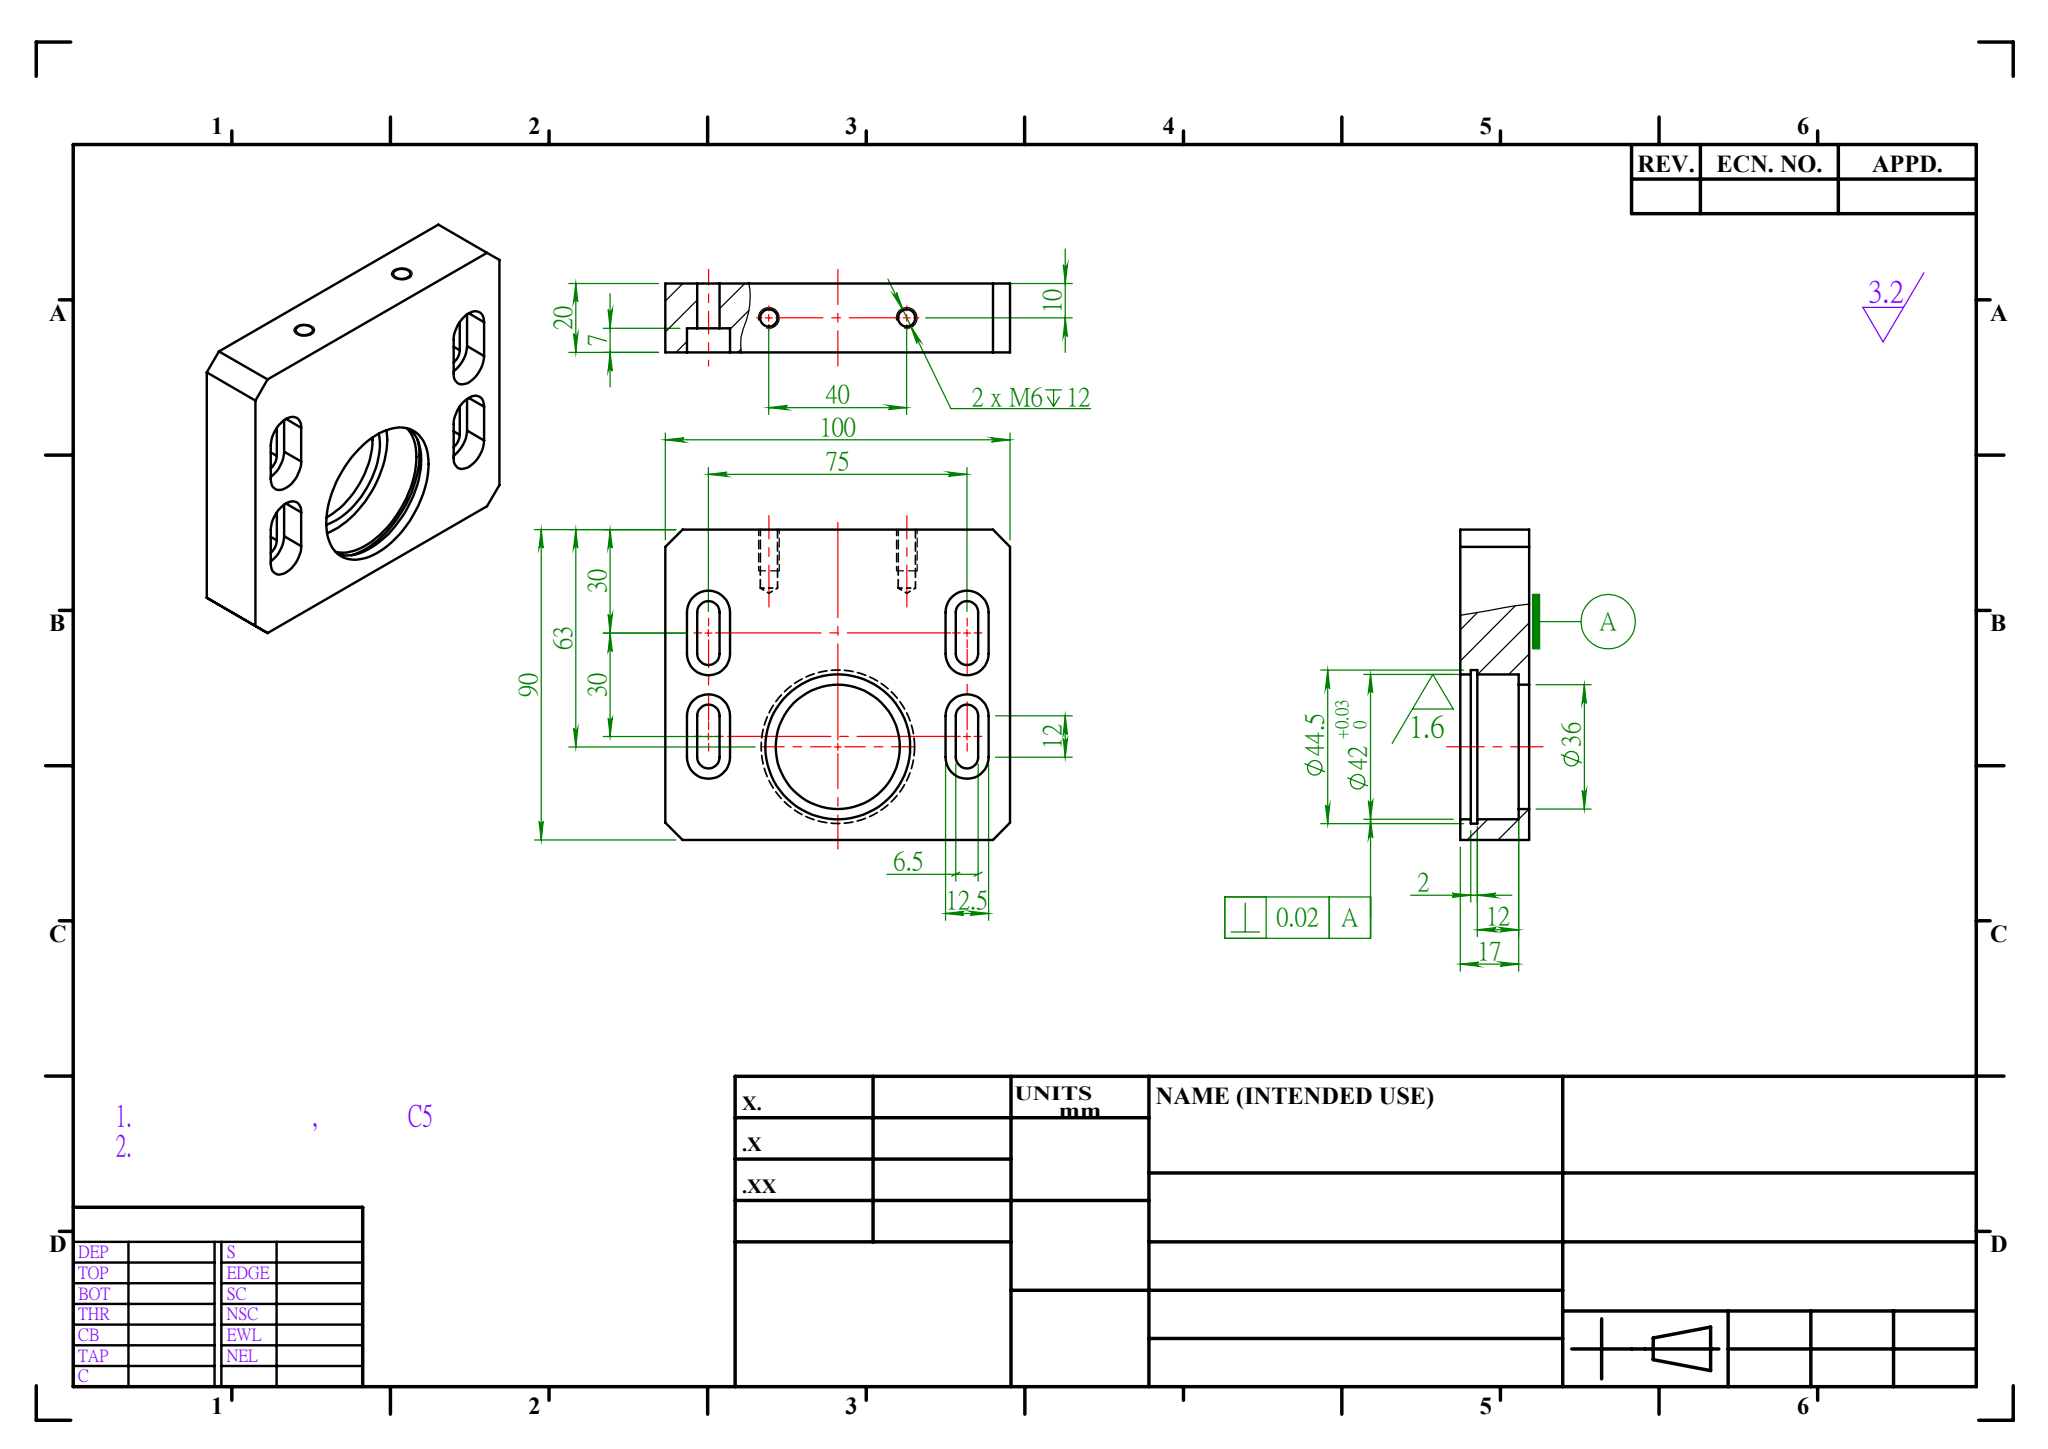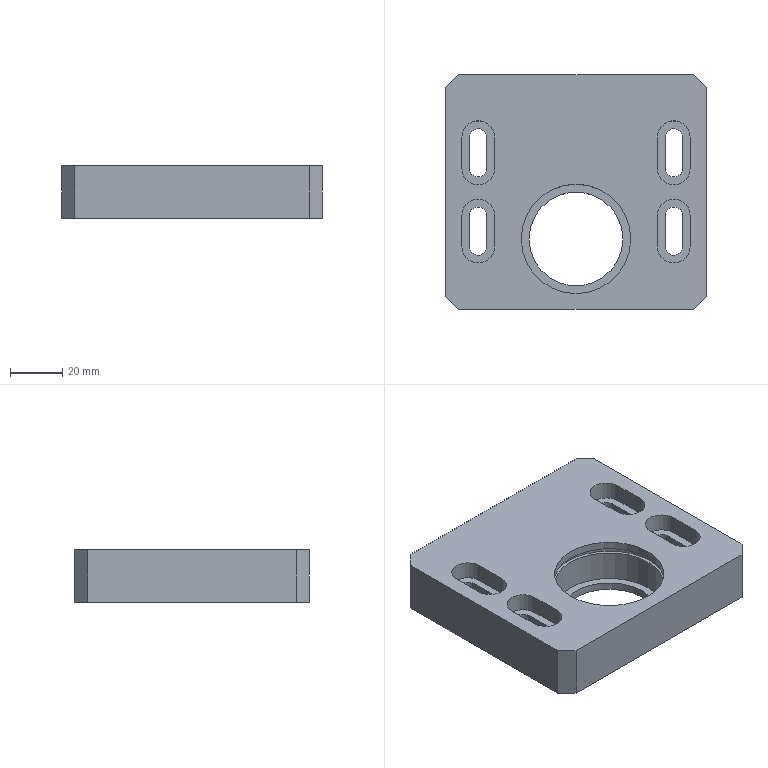Part | SolidWorks | mm | 1 solid | 65 faces | box 100 x 90 x 20 mm | volume 137958 mm3 | plane 33 | cylinder 28 | cone 4 | commonest cylinder face diameters 6.5 x8 12.5 x8 5 x4 42 x4 44.5 x2 36 x2
build123d program:
from build123d import *

# Parameters (mm, degrees)
SKETCH1_W             = 100
SKETCH1_H             = 90
BOSS_EXTRUDE1_DEPTH   = 20
SKETCH2_3_R           = 18
CUT_EXTRUDE1_DEPTH    = 83.879
SKETCH2_3_2_R         = 21
CUT_EXTRUDE2_DEPTH    = 17
SKETCH3_R             = 22.25
CUT_EXTRUDE3_DEPTH    = 1.95
CUT_EXTRUDE4_DEPTH    = 83.879
CUT_EXTRUDE5_DEPTH    = 7
CHAMFER1_SIZE         = 5
M6_TAPPED_HOLE1_D     = 5
M6_TAPPED_HOLE1_DEPTH = 17
M6_TAPPED_HOLE1_TIP   = 1.502


with BuildPart() as part:
    # Sketch1 → Boss-Extrude1 (new body)
    with BuildSketch(Plane.XY):
        with Locations((0, 18)):
            Rectangle(SKETCH1_W, SKETCH1_H)
    extrude(amount=BOSS_EXTRUDE1_DEPTH)

    # Sketch2_3 → Cut-Extrude1 (cut, through all)
    with BuildSketch(Plane.XY.offset(20)):
        Circle(SKETCH2_3_R)
    extrude(amount=-CUT_EXTRUDE1_DEPTH, mode=Mode.SUBTRACT)

    # Sketch2_3 2 → Cut-Extrude2 (cut)
    with BuildSketch(Plane.XY.offset(20)):
        Circle(SKETCH2_3_2_R)
    extrude(amount=-CUT_EXTRUDE2_DEPTH, mode=Mode.SUBTRACT)

    # Sketch3 → Cut-Extrude3 (cut)
    with BuildSketch(Plane.XY.offset(15)):
        Circle(SKETCH3_R)
    extrude(amount=CUT_EXTRUDE3_DEPTH, mode=Mode.SUBTRACT)

    # Sketch4_3 → Cut-Extrude4 (cut, through all)
    with BuildSketch(Plane.XY.offset(20)):
        with BuildLine():
            Line((-40.75, 39), (-40.75, 27))
            ThreePointArc((-40.75, 27), (-37.5, 23.75), (-34.25, 27))
            Line((-34.25, 27), (-34.25, 39))
            ThreePointArc((-34.25, 39), (-37.5, 42.25), (-40.75, 39))
        make_face()
        with BuildLine():
            Line((34.25, 9), (34.25, -3))
            ThreePointArc((34.25, -3), (37.5, -6.25), (40.75, -3))
            Line((40.75, -3), (40.75, 9))
            ThreePointArc((40.75, 9), (37.5, 12.25), (34.25, 9))
        make_face()
        with BuildLine():
            Line((34.25, 39), (34.25, 27))
            ThreePointArc((34.25, 27), (37.5, 23.75), (40.75, 27))
            Line((40.75, 27), (40.75, 39))
            ThreePointArc((40.75, 39), (37.5, 42.25), (34.25, 39))
        make_face()
        with BuildLine():
            Line((-40.75, 9), (-40.75, -3))
            ThreePointArc((-40.75, -3), (-37.5, -6.25), (-34.25, -3))
            Line((-34.25, -3), (-34.25, 9))
            ThreePointArc((-34.25, 9), (-37.5, 12.25), (-40.75, 9))
        make_face()
    extrude(amount=-CUT_EXTRUDE4_DEPTH, mode=Mode.SUBTRACT)

    # Sketch4_3 2 → Cut-Extrude5 (cut)
    # profile 1 of 4: a face of its own
    with BuildSketch(Plane.XY.offset(20)):
        with BuildLine():
            Line((-31.25, 9), (-31.25, -3))
            ThreePointArc((-31.25, -3), (-37.5, -9.25), (-43.75, -3))
            Line((-43.75, -3), (-43.75, 9))
            ThreePointArc((-43.75, 9), (-37.5, 15.25), (-31.25, 9))
        make_face()
        with BuildLine():
            ThreePointArc((-40.75, -3), (-37.5, -6.25), (-34.25, -3))
            Line((-34.25, -3), (-34.25, 9))
            ThreePointArc((-34.25, 9), (-37.5, 12.25), (-40.75, 9))
            Line((-40.75, 9), (-40.75, -3))
        make_face(mode=Mode.SUBTRACT)
    # profile 2 of 4: a face of its own
    with BuildSketch(Plane.XY.offset(20)):
        with BuildLine():
            Line((43.75, 39), (43.75, 27))
            ThreePointArc((43.75, 27), (37.5, 20.75), (31.25, 27))
            Line((31.25, 27), (31.25, 39))
            ThreePointArc((31.25, 39), (37.5, 45.25), (43.75, 39))
        make_face()
        with BuildLine():
            ThreePointArc((34.25, 27), (37.5, 23.75), (40.75, 27))
            Line((40.75, 27), (40.75, 39))
            ThreePointArc((40.75, 39), (37.5, 42.25), (34.25, 39))
            Line((34.25, 39), (34.25, 27))
        make_face(mode=Mode.SUBTRACT)
    # profile 3 of 4: a face of its own
    with BuildSketch(Plane.XY.offset(20)):
        with BuildLine():
            Line((43.75, 9), (43.75, -3))
            ThreePointArc((43.75, -3), (37.5, -9.25), (31.25, -3))
            Line((31.25, -3), (31.25, 9))
            ThreePointArc((31.25, 9), (37.5, 15.25), (43.75, 9))
        make_face()
        with BuildLine():
            ThreePointArc((34.25, -3), (37.5, -6.25), (40.75, -3))
            Line((40.75, -3), (40.75, 9))
            ThreePointArc((40.75, 9), (37.5, 12.25), (34.25, 9))
            Line((34.25, 9), (34.25, -3))
        make_face(mode=Mode.SUBTRACT)
    # profile 4 of 4: a face of its own
    with BuildSketch(Plane.XY.offset(20)):
        with BuildLine():
            Line((-43.75, 39), (-43.75, 27))
            ThreePointArc((-43.75, 27), (-37.5, 20.75), (-31.25, 27))
            Line((-31.25, 27), (-31.25, 39))
            ThreePointArc((-31.25, 39), (-37.5, 45.25), (-43.75, 39))
        make_face()
    extrude(amount=-CUT_EXTRUDE5_DEPTH, mode=Mode.SUBTRACT)

    # Chamfer1
    chamfer1_edges = [part.edges().sort_by_distance(p)[0] for p in [
        (-50, 63, 10),
        (50, 63, 10),
        (50, -27, 10),
        (-50, -27, 10),
    ]]
    chamfer(chamfer1_edges, length=CHAMFER1_SIZE)

    # M6 Tapped Hole1
    with Locations(Plane(origin=(0, 63, 0), x_dir=(1, 0, 0), z_dir=(0, 1, 0))):
        with Locations((-20, -10), (20, -10)):
            Hole(M6_TAPPED_HOLE1_D / 2, depth=M6_TAPPED_HOLE1_DEPTH)
            with Locations((0, 0, -(M6_TAPPED_HOLE1_DEPTH + M6_TAPPED_HOLE1_TIP / 2))):  # 118° drill point
                Cone(0, M6_TAPPED_HOLE1_D / 2, M6_TAPPED_HOLE1_TIP, mode=Mode.SUBTRACT)


solid = part.part